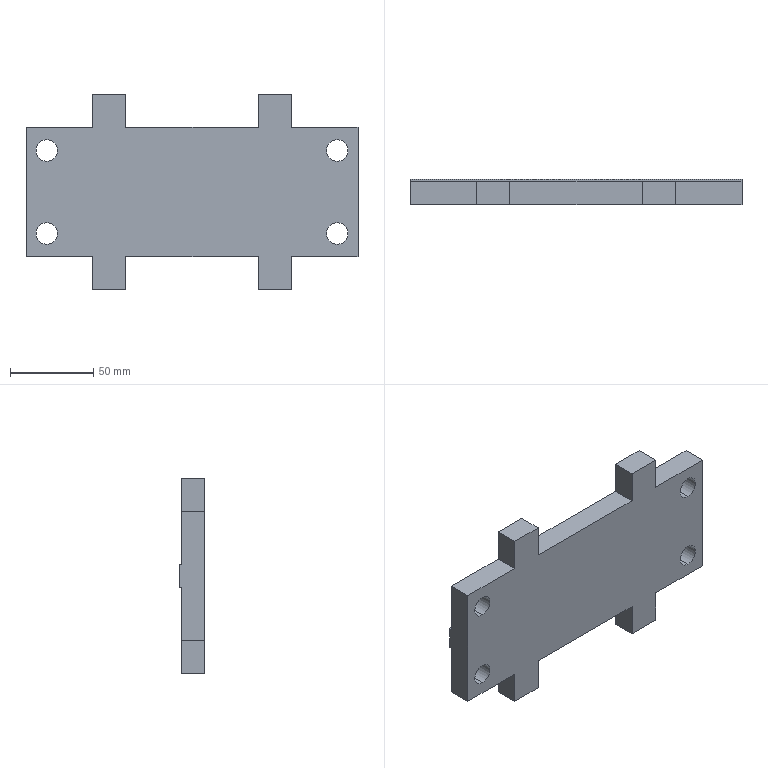Component | SolidWorks | NewTypeCurveBenderReinforcementSeatUpperWheelBox2-DoubleWheel-1 | 1 solid | 34 faces | box 200 x 15.5 x 118 mm | volume 237567 mm3 | plane 26 | cylinder 8 | commonest cylinder face diameters 13 x8
build123d program:
from build123d import *

# Parameters (mm, degrees)
SKETCH1_W           = 200
SKETCH1_H           = 78
BOSS_EXTRUDE1_DEPTH = 14
SKETCH2_W           = 20
SKETCH2_H           = 20
BOSS_EXTRUDE2_DEPTH = 14
SKETCH3_R           = 6.5
CUT_EXTRUDE1_DEPTH  = 30
SKETCH5_W           = 14
SKETCH5_H           = 1.5
BOSS_EXTRUDE3_DEPTH = 200


with BuildPart() as part:
    # Sketch1 → Boss-Extrude1 (new body)
    with BuildSketch(Plane(origin=(0, 0, 0), x_dir=(1, 0, 0), z_dir=(0, 1, 0))):
        Rectangle(SKETCH1_W, SKETCH1_H)
    extrude(amount=BOSS_EXTRUDE1_DEPTH)

    # Sketch2 → Boss-Extrude2 (add)
    with BuildSketch(Plane(origin=(0, 14, 0), x_dir=(1, 0, 0), z_dir=(0, 1, 0))):
        with Locations((-50, -49)):
            Rectangle(SKETCH2_W, SKETCH2_H)
        with Locations((-50, 49)):
            Rectangle(SKETCH2_W, SKETCH2_H)
        with Locations((50, -49)):
            Rectangle(SKETCH2_W, SKETCH2_H)
        with Locations((50, 49)):
            Rectangle(SKETCH2_W, SKETCH2_H)
    extrude(amount=-BOSS_EXTRUDE2_DEPTH)

    # Sketch3 → Cut-Extrude1 (cut)
    with BuildSketch(Plane(origin=(0, 14, 0), x_dir=(1, 0, 0), z_dir=(0, 1, 0))):
        with Locations(Location((-87.5, 25, 0), (0, 0, 270))):
            Circle(SKETCH3_R)
        with Locations(Location((87.5, 25, 0), (0, 0, 270))):
            Circle(SKETCH3_R)
        with Locations(Location((87.5, -25, 0), (0, 0, 270))):
            Circle(SKETCH3_R)
        with Locations(Location((-87.5, -25, 0), (0, 0, 270))):
            Circle(SKETCH3_R)
    extrude(amount=-CUT_EXTRUDE1_DEPTH, mode=Mode.SUBTRACT)

    # Sketch5 → Boss-Extrude3 (add)
    with BuildSketch(Plane(origin=(100, 0, 0), x_dir=(0, 0, -1), z_dir=(1, 0, 0))):
        with Locations((0, -0.75)):
            Rectangle(SKETCH5_W, SKETCH5_H)
    extrude(amount=-BOSS_EXTRUDE3_DEPTH)


solid = part.part

# Placed as in the assembly
solid = solid.moved(Location((0, -133, 0), (180, 0, 0)))
STEP:
#1=COLOUR_RGB('',0.7922,0.8196,0.9333);
#2=FILL_AREA_STYLE_COLOUR('',#1);
#3=FILL_AREA_STYLE('',(#2));
#4=SURFACE_STYLE_FILL_AREA(#3);
#5=SURFACE_SIDE_STYLE('',(#4));
#6=SURFACE_STYLE_USAGE(.BOTH.,#5);
#7=PRESENTATION_STYLE_ASSIGNMENT((#6));
#8=CARTESIAN_POINT('',(3.445,-5.236,0.7283));
#9=VERTEX_POINT('',#8);
#10=CARTESIAN_POINT('',(3.445,-5.236,1.24));
#11=VERTEX_POINT('',#10);
#12=CARTESIAN_POINT('',(3.445,-5.236,0.9843));
#13=DIRECTION('',(0.,-1.,-0.));
#14=DIRECTION('',(0.,0.,1.));
#15=AXIS2_PLACEMENT_3D('',#12,#13,#14);
#16=CIRCLE('',#15,0.2559);
#17=EDGE_CURVE('',#9,#11,#16,.T.);
#18=ORIENTED_EDGE('',*,*,#17,.F.);
#19=CARTESIAN_POINT('',(3.445,-5.787,0.7283));
#20=VERTEX_POINT('',#19);
#21=CARTESIAN_POINT('',(3.445,-4.606,0.7283));
#22=DIRECTION('',(0.,-1.,-0.));
#23=VECTOR('',#22,39.37);
#24=LINE('',#21,#23);
#25=EDGE_CURVE('',#9,#20,#24,.T.);
#26=ORIENTED_EDGE('',*,*,#25,.T.);
#27=CARTESIAN_POINT('',(3.445,-5.787,1.24));
#28=VERTEX_POINT('',#27);
#29=CARTESIAN_POINT('',(3.445,-5.787,0.9843));
#30=DIRECTION('',(0.,-1.,-0.));
#31=DIRECTION('',(0.,0.,-1.));
#32=AXIS2_PLACEMENT_3D('',#29,#30,#31);
#33=CIRCLE('',#32,0.2559);
#34=EDGE_CURVE('',#20,#28,#33,.T.);
#35=ORIENTED_EDGE('',*,*,#34,.T.);
#36=CARTESIAN_POINT('',(3.445,-4.606,1.24));
#37=DIRECTION('',(0.,-1.,-0.));
#38=VECTOR('',#37,39.37);
#39=LINE('',#36,#38);
#40=EDGE_CURVE('',#11,#28,#39,.T.);
#41=ORIENTED_EDGE('',*,*,#40,.F.);
#42=EDGE_LOOP('',(#18,#26,#35,#41));
#43=FACE_OUTER_BOUND('',#42,.T.);
#44=CARTESIAN_POINT('',(3.445,-4.606,0.9843));
#45=DIRECTION('',(0.,-1.,-0.));
#46=DIRECTION('',(0.,0.,1.));
#47=AXIS2_PLACEMENT_3D('',#44,#45,#46);
#48=CYLINDRICAL_SURFACE('',#47,0.2559);
#49=ADVANCED_FACE('',(#43),#48,.F.);
#50=CARTESIAN_POINT('',(-3.445,-5.236,0.7283));
#51=VERTEX_POINT('',#50);
#52=CARTESIAN_POINT('',(-3.445,-5.236,1.24));
#53=VERTEX_POINT('',#52);
#54=CARTESIAN_POINT('',(-3.445,-5.236,0.9843));
#55=DIRECTION('',(0.,-1.,-0.));
#56=DIRECTION('',(0.,0.,1.));
#57=AXIS2_PLACEMENT_3D('',#54,#55,#56);
#58=CIRCLE('',#57,0.2559);
#59=EDGE_CURVE('',#51,#53,#58,.T.);
#60=ORIENTED_EDGE('',*,*,#59,.F.);
#61=CARTESIAN_POINT('',(-3.445,-5.787,0.7283));
#62=VERTEX_POINT('',#61);
#63=CARTESIAN_POINT('',(-3.445,-4.606,0.7283));
#64=DIRECTION('',(0.,-1.,-0.));
#65=VECTOR('',#64,39.37);
#66=LINE('',#63,#65);
#67=EDGE_CURVE('',#51,#62,#66,.T.);
#68=ORIENTED_EDGE('',*,*,#67,.T.);
#69=CARTESIAN_POINT('',(-3.445,-5.787,1.24));
#70=VERTEX_POINT('',#69);
#71=CARTESIAN_POINT('',(-3.445,-5.787,0.9843));
#72=DIRECTION('',(0.,-1.,-0.));
#73=DIRECTION('',(0.,0.,1.));
#74=AXIS2_PLACEMENT_3D('',#71,#72,#73);
#75=CIRCLE('',#74,0.2559);
#76=EDGE_CURVE('',#62,#70,#75,.T.);
#77=ORIENTED_EDGE('',*,*,#76,.T.);
#78=CARTESIAN_POINT('',(-3.445,-4.606,1.24));
#79=DIRECTION('',(0.,-1.,-0.));
#80=VECTOR('',#79,39.37);
#81=LINE('',#78,#80);
#82=EDGE_CURVE('',#53,#70,#81,.T.);
#83=ORIENTED_EDGE('',*,*,#82,.F.);
#84=EDGE_LOOP('',(#60,#68,#77,#83));
#85=FACE_OUTER_BOUND('',#84,.T.);
#86=CARTESIAN_POINT('',(-3.445,-4.606,0.9843));
#87=DIRECTION('',(0.,-1.,-0.));
#88=DIRECTION('',(0.,0.,1.));
#89=AXIS2_PLACEMENT_3D('',#86,#87,#88);
#90=CYLINDRICAL_SURFACE('',#89,0.2559);
#91=ADVANCED_FACE('',(#85),#90,.F.);
#92=CARTESIAN_POINT('',(-3.445,-5.236,-1.24));
#93=VERTEX_POINT('',#92);
#94=CARTESIAN_POINT('',(-3.445,-5.236,-0.7283));
#95=VERTEX_POINT('',#94);
#96=CARTESIAN_POINT('',(-3.445,-5.236,-0.9843));
#97=DIRECTION('',(0.,-1.,-0.));
#98=DIRECTION('',(0.,0.,1.));
#99=AXIS2_PLACEMENT_3D('',#96,#97,#98);
#100=CIRCLE('',#99,0.2559);
#101=EDGE_CURVE('',#93,#95,#100,.T.);
#102=ORIENTED_EDGE('',*,*,#101,.F.);
#103=CARTESIAN_POINT('',(-3.445,-5.787,-1.24));
#104=VERTEX_POINT('',#103);
#105=CARTESIAN_POINT('',(-3.445,-4.606,-1.24));
#106=DIRECTION('',(0.,-1.,-0.));
#107=VECTOR('',#106,39.37);
#108=LINE('',#105,#107);
#109=EDGE_CURVE('',#93,#104,#108,.T.);
#110=ORIENTED_EDGE('',*,*,#109,.T.);
#111=CARTESIAN_POINT('',(-3.445,-5.787,-0.7283));
#112=VERTEX_POINT('',#111);
#113=CARTESIAN_POINT('',(-3.445,-5.787,-0.9843));
#114=DIRECTION('',(0.,-1.,-0.));
#115=DIRECTION('',(0.,0.,-1.));
#116=AXIS2_PLACEMENT_3D('',#113,#114,#115);
#117=CIRCLE('',#116,0.2559);
#118=EDGE_CURVE('',#104,#112,#117,.T.);
#119=ORIENTED_EDGE('',*,*,#118,.T.);
#120=CARTESIAN_POINT('',(-3.445,-4.606,-0.7283));
#121=DIRECTION('',(0.,-1.,-0.));
#122=VECTOR('',#121,39.37);
#123=LINE('',#120,#122);
#124=EDGE_CURVE('',#95,#112,#123,.T.);
#125=ORIENTED_EDGE('',*,*,#124,.F.);
#126=EDGE_LOOP('',(#102,#110,#119,#125));
#127=FACE_OUTER_BOUND('',#126,.T.);
#128=CARTESIAN_POINT('',(-3.445,-4.606,-0.9843));
#129=DIRECTION('',(0.,-1.,-0.));
#130=DIRECTION('',(0.,0.,1.));
#131=AXIS2_PLACEMENT_3D('',#128,#129,#130);
#132=CYLINDRICAL_SURFACE('',#131,0.2559);
#133=ADVANCED_FACE('',(#127),#132,.F.);
#134=CARTESIAN_POINT('',(3.445,-5.236,-1.24));
#135=VERTEX_POINT('',#134);
#136=CARTESIAN_POINT('',(3.445,-5.236,-0.7283));
#137=VERTEX_POINT('',#136);
#138=CARTESIAN_POINT('',(3.445,-5.236,-0.9843));
#139=DIRECTION('',(0.,-1.,-0.));
#140=DIRECTION('',(0.,0.,1.));
#141=AXIS2_PLACEMENT_3D('',#138,#139,#140);
#142=CIRCLE('',#141,0.2559);
#143=EDGE_CURVE('',#135,#137,#142,.T.);
#144=ORIENTED_EDGE('',*,*,#143,.F.);
#145=CARTESIAN_POINT('',(3.445,-5.787,-1.24));
#146=VERTEX_POINT('',#145);
#147=CARTESIAN_POINT('',(3.445,-4.606,-1.24));
#148=DIRECTION('',(0.,-1.,-0.));
#149=VECTOR('',#148,39.37);
#150=LINE('',#147,#149);
#151=EDGE_CURVE('',#135,#146,#150,.T.);
#152=ORIENTED_EDGE('',*,*,#151,.T.);
#153=CARTESIAN_POINT('',(3.445,-5.787,-0.7283));
#154=VERTEX_POINT('',#153);
#155=CARTESIAN_POINT('',(3.445,-5.787,-0.9843));
#156=DIRECTION('',(0.,-1.,-0.));
#157=DIRECTION('',(0.,0.,1.));
#158=AXIS2_PLACEMENT_3D('',#155,#156,#157);
#159=CIRCLE('',#158,0.2559);
#160=EDGE_CURVE('',#146,#154,#159,.T.);
#161=ORIENTED_EDGE('',*,*,#160,.T.);
#162=CARTESIAN_POINT('',(3.445,-4.606,-0.7283));
#163=DIRECTION('',(0.,-1.,-0.));
#164=VECTOR('',#163,39.37);
#165=LINE('',#162,#164);
#166=EDGE_CURVE('',#137,#154,#165,.T.);
#167=ORIENTED_EDGE('',*,*,#166,.F.);
#168=EDGE_LOOP('',(#144,#152,#161,#167));
#169=FACE_OUTER_BOUND('',#168,.T.);
#170=CARTESIAN_POINT('',(3.445,-4.606,-0.9843));
#171=DIRECTION('',(0.,-1.,-0.));
#172=DIRECTION('',(0.,0.,1.));
#173=AXIS2_PLACEMENT_3D('',#170,#171,#172);
#174=CYLINDRICAL_SURFACE('',#173,0.2559);
#175=ADVANCED_FACE('',(#169),#174,.F.);
#176=CARTESIAN_POINT('',(3.445,-5.236,-0.9843));
#177=DIRECTION('',(0.,-1.,-0.));
#178=DIRECTION('',(0.,0.,1.));
#179=AXIS2_PLACEMENT_3D('',#176,#177,#178);
#180=CIRCLE('',#179,0.2559);
#181=EDGE_CURVE('',#137,#135,#180,.T.);
#182=ORIENTED_EDGE('',*,*,#181,.T.);
#183=ORIENTED_EDGE('',*,*,#143,.T.);
#184=EDGE_LOOP('',(#182,#183));
#185=FACE_BOUND('',#184,.T.);
#186=CARTESIAN_POINT('',(-3.445,-5.236,-0.9843));
#187=DIRECTION('',(0.,-1.,-0.));
#188=DIRECTION('',(0.,0.,1.));
#189=AXIS2_PLACEMENT_3D('',#186,#187,#188);
#190=CIRCLE('',#189,0.2559);
#191=EDGE_CURVE('',#95,#93,#190,.T.);
#192=ORIENTED_EDGE('',*,*,#191,.T.);
#193=ORIENTED_EDGE('',*,*,#101,.T.);
#194=EDGE_LOOP('',(#192,#193));
#195=FACE_BOUND('',#194,.T.);
#196=CARTESIAN_POINT('',(3.937,-5.236,-0.2756));
#197=VERTEX_POINT('',#196);
#198=CARTESIAN_POINT('',(-3.937,-5.236,-0.2756));
#199=VERTEX_POINT('',#198);
#200=CARTESIAN_POINT('',(4.491,-5.236,-0.2756));
#201=DIRECTION('',(-1.,-0.,0.));
#202=VECTOR('',#201,39.37);
#203=LINE('',#200,#202);
#204=EDGE_CURVE('',#197,#199,#203,.T.);
#205=ORIENTED_EDGE('',*,*,#204,.F.);
#206=CARTESIAN_POINT('',(3.937,-5.236,-1.535));
#207=VERTEX_POINT('',#206);
#208=CARTESIAN_POINT('',(3.937,-5.236,-1.535));
#209=DIRECTION('',(0.,0.,1.));
#210=VECTOR('',#209,39.37);
#211=LINE('',#208,#210);
#212=EDGE_CURVE('',#207,#197,#211,.T.);
#213=ORIENTED_EDGE('',*,*,#212,.F.);
#214=CARTESIAN_POINT('',(2.362,-5.236,-1.535));
#215=VERTEX_POINT('',#214);
#216=CARTESIAN_POINT('',(3.937,-5.236,-1.535));
#217=DIRECTION('',(1.,0.,0.));
#218=VECTOR('',#217,39.37);
#219=LINE('',#216,#218);
#220=EDGE_CURVE('',#215,#207,#219,.T.);
#221=ORIENTED_EDGE('',*,*,#220,.F.);
#222=CARTESIAN_POINT('',(2.362,-5.236,-2.323));
#223=VERTEX_POINT('',#222);
#224=CARTESIAN_POINT('',(2.362,-5.236,-1.535));
#225=DIRECTION('',(0.,-0.,-1.));
#226=VECTOR('',#225,39.37);
#227=LINE('',#224,#226);
#228=EDGE_CURVE('',#215,#223,#227,.T.);
#229=ORIENTED_EDGE('',*,*,#228,.T.);
#230=CARTESIAN_POINT('',(1.575,-5.236,-2.323));
#231=VERTEX_POINT('',#230);
#232=CARTESIAN_POINT('',(2.362,-5.236,-2.323));
#233=DIRECTION('',(-1.,-0.,0.));
#234=VECTOR('',#233,39.37);
#235=LINE('',#232,#234);
#236=EDGE_CURVE('',#223,#231,#235,.T.);
#237=ORIENTED_EDGE('',*,*,#236,.T.);
#238=CARTESIAN_POINT('',(1.575,-5.236,-1.535));
#239=VERTEX_POINT('',#238);
#240=CARTESIAN_POINT('',(1.575,-5.236,-1.535));
#241=DIRECTION('',(0.,0.,1.));
#242=VECTOR('',#241,39.37);
#243=LINE('',#240,#242);
#244=EDGE_CURVE('',#231,#239,#243,.T.);
#245=ORIENTED_EDGE('',*,*,#244,.T.);
#246=CARTESIAN_POINT('',(-1.575,-5.236,-1.535));
#247=VERTEX_POINT('',#246);
#248=CARTESIAN_POINT('',(3.937,-5.236,-1.535));
#249=DIRECTION('',(1.,0.,0.));
#250=VECTOR('',#249,39.37);
#251=LINE('',#248,#250);
#252=EDGE_CURVE('',#247,#239,#251,.T.);
#253=ORIENTED_EDGE('',*,*,#252,.F.);
#254=CARTESIAN_POINT('',(-1.575,-5.236,-2.323));
#255=VERTEX_POINT('',#254);
#256=CARTESIAN_POINT('',(-1.575,-5.236,-1.535));
#257=DIRECTION('',(-0.,-0.,-1.));
#258=VECTOR('',#257,39.37);
#259=LINE('',#256,#258);
#260=EDGE_CURVE('',#247,#255,#259,.T.);
#261=ORIENTED_EDGE('',*,*,#260,.T.);
#262=CARTESIAN_POINT('',(-2.362,-5.236,-2.323));
#263=VERTEX_POINT('',#262);
#264=CARTESIAN_POINT('',(-2.362,-5.236,-2.323));
#265=DIRECTION('',(-1.,-0.,-0.));
#266=VECTOR('',#265,39.37);
#267=LINE('',#264,#266);
#268=EDGE_CURVE('',#255,#263,#267,.T.);
#269=ORIENTED_EDGE('',*,*,#268,.T.);
#270=CARTESIAN_POINT('',(-2.362,-5.236,-1.535));
#271=VERTEX_POINT('',#270);
#272=CARTESIAN_POINT('',(-2.362,-5.236,-1.535));
#273=DIRECTION('',(0.,0.,1.));
#274=VECTOR('',#273,39.37);
#275=LINE('',#272,#274);
#276=EDGE_CURVE('',#263,#271,#275,.T.);
#277=ORIENTED_EDGE('',*,*,#276,.T.);
#278=CARTESIAN_POINT('',(-3.937,-5.236,-1.535));
#279=VERTEX_POINT('',#278);
#280=CARTESIAN_POINT('',(3.937,-5.236,-1.535));
#281=DIRECTION('',(1.,0.,0.));
#282=VECTOR('',#281,39.37);
#283=LINE('',#280,#282);
#284=EDGE_CURVE('',#279,#271,#283,.T.);
#285=ORIENTED_EDGE('',*,*,#284,.F.);
#286=CARTESIAN_POINT('',(-3.937,-5.236,-1.535));
#287=DIRECTION('',(-0.,-0.,-1.));
#288=VECTOR('',#287,39.37);
#289=LINE('',#286,#288);
#290=EDGE_CURVE('',#199,#279,#289,.T.);
#291=ORIENTED_EDGE('',*,*,#290,.F.);
#292=EDGE_LOOP('',(#205,#213,#221,#229,#237,#245,#253,#261,#269,#277,#285,#291));
#293=FACE_OUTER_BOUND('',#292,.T.);
#294=CARTESIAN_POINT('',(-0.,-5.236,0.));
#295=DIRECTION('',(0.,-1.,0.));
#296=DIRECTION('',(0.,0.,1.));
#297=AXIS2_PLACEMENT_3D('',#294,#295,#296);
#298=PLANE('',#297);
#299=ADVANCED_FACE('',(#185,#195,#293),#298,.F.);
#300=CARTESIAN_POINT('',(-1.575,-5.787,-1.535));
#301=VERTEX_POINT('',#300);
#302=CARTESIAN_POINT('',(1.575,-5.787,-1.535));
#303=VERTEX_POINT('',#302);
#304=CARTESIAN_POINT('',(3.937,-5.787,-1.535));
#305=DIRECTION('',(1.,0.,0.));
#306=VECTOR('',#305,39.37);
#307=LINE('',#304,#306);
#308=EDGE_CURVE('',#301,#303,#307,.T.);
#309=ORIENTED_EDGE('',*,*,#308,.F.);
#310=CARTESIAN_POINT('',(-1.575,-4.123,-1.535));
#311=DIRECTION('',(0.,-1.,-0.));
#312=VECTOR('',#311,39.37);
#313=LINE('',#310,#312);
#314=EDGE_CURVE('',#247,#301,#313,.T.);
#315=ORIENTED_EDGE('',*,*,#314,.F.);
#316=ORIENTED_EDGE('',*,*,#252,.T.);
#317=CARTESIAN_POINT('',(1.575,-4.123,-1.535));
#318=DIRECTION('',(0.,-1.,-0.));
#319=VECTOR('',#318,39.37);
#320=LINE('',#317,#319);
#321=EDGE_CURVE('',#239,#303,#320,.T.);
#322=ORIENTED_EDGE('',*,*,#321,.T.);
#323=EDGE_LOOP('',(#309,#315,#316,#322));
#324=FACE_OUTER_BOUND('',#323,.T.);
#325=CARTESIAN_POINT('',(3.937,-5.787,-1.535));
#326=DIRECTION('',(-0.,0.,1.));
#327=DIRECTION('',(-1.,-0.,0.));
#328=AXIS2_PLACEMENT_3D('',#325,#326,#327);
#329=PLANE('',#328);
#330=ADVANCED_FACE('',(#324),#329,.F.);
#331=CARTESIAN_POINT('',(-2.362,-5.787,1.535));
#332=VERTEX_POINT('',#331);
#333=CARTESIAN_POINT('',(-3.937,-5.787,1.535));
#334=VERTEX_POINT('',#333);
#335=CARTESIAN_POINT('',(3.937,-5.787,1.535));
#336=DIRECTION('',(-1.,-0.,0.));
#337=VECTOR('',#336,39.37);
#338=LINE('',#335,#337);
#339=EDGE_CURVE('',#332,#334,#338,.T.);
#340=ORIENTED_EDGE('',*,*,#339,.F.);
#341=CARTESIAN_POINT('',(-2.362,-5.236,1.535));
#342=VERTEX_POINT('',#341);
#343=CARTESIAN_POINT('',(-2.362,-4.123,1.535));
#344=DIRECTION('',(0.,-1.,-0.));
#345=VECTOR('',#344,39.37);
#346=LINE('',#343,#345);
#347=EDGE_CURVE('',#342,#332,#346,.T.);
#348=ORIENTED_EDGE('',*,*,#347,.F.);
#349=CARTESIAN_POINT('',(-3.937,-5.236,1.535));
#350=VERTEX_POINT('',#349);
#351=CARTESIAN_POINT('',(3.937,-5.236,1.535));
#352=DIRECTION('',(-1.,-0.,0.));
#353=VECTOR('',#352,39.37);
#354=LINE('',#351,#353);
#355=EDGE_CURVE('',#342,#350,#354,.T.);
#356=ORIENTED_EDGE('',*,*,#355,.T.);
#357=CARTESIAN_POINT('',(-3.937,-5.787,1.535));
#358=DIRECTION('',(-0.,1.,0.));
#359=VECTOR('',#358,39.37);
#360=LINE('',#357,#359);
#361=EDGE_CURVE('',#334,#350,#360,.T.);
#362=ORIENTED_EDGE('',*,*,#361,.F.);
#363=EDGE_LOOP('',(#340,#348,#356,#362));
#364=FACE_OUTER_BOUND('',#363,.T.);
#365=CARTESIAN_POINT('',(3.937,-5.787,1.535));
#366=DIRECTION('',(0.,-0.,-1.));
#367=DIRECTION('',(1.,0.,0.));
#368=AXIS2_PLACEMENT_3D('',#365,#366,#367);
#369=PLANE('',#368);
#370=ADVANCED_FACE('',(#364),#369,.F.);
#371=CARTESIAN_POINT('',(1.575,-5.236,1.535));
#372=VERTEX_POINT('',#371);
#373=CARTESIAN_POINT('',(-1.575,-5.236,1.535));
#374=VERTEX_POINT('',#373);
#375=CARTESIAN_POINT('',(3.937,-5.236,1.535));
#376=DIRECTION('',(-1.,-0.,0.));
#377=VECTOR('',#376,39.37);
#378=LINE('',#375,#377);
#379=EDGE_CURVE('',#372,#374,#378,.T.);
#380=ORIENTED_EDGE('',*,*,#379,.T.);
#381=CARTESIAN_POINT('',(-1.575,-5.787,1.535));
#382=VERTEX_POINT('',#381);
#383=CARTESIAN_POINT('',(-1.575,-4.123,1.535));
#384=DIRECTION('',(0.,-1.,-0.));
#385=VECTOR('',#384,39.37);
#386=LINE('',#383,#385);
#387=EDGE_CURVE('',#374,#382,#386,.T.);
#388=ORIENTED_EDGE('',*,*,#387,.T.);
#389=CARTESIAN_POINT('',(1.575,-5.787,1.535));
#390=VERTEX_POINT('',#389);
#391=CARTESIAN_POINT('',(3.937,-5.787,1.535));
#392=DIRECTION('',(-1.,-0.,0.));
#393=VECTOR('',#392,39.37);
#394=LINE('',#391,#393);
#395=EDGE_CURVE('',#390,#382,#394,.T.);
#396=ORIENTED_EDGE('',*,*,#395,.F.);
#397=CARTESIAN_POINT('',(1.575,-4.123,1.535));
#398=DIRECTION('',(0.,-1.,-0.));
#399=VECTOR('',#398,39.37);
#400=LINE('',#397,#399);
#401=EDGE_CURVE('',#372,#390,#400,.T.);
#402=ORIENTED_EDGE('',*,*,#401,.F.);
#403=EDGE_LOOP('',(#380,#388,#396,#402));
#404=FACE_OUTER_BOUND('',#403,.T.);
#405=CARTESIAN_POINT('',(3.937,-5.787,1.535));
#406=DIRECTION('',(0.,-0.,-1.));
#407=DIRECTION('',(1.,0.,0.));
#408=AXIS2_PLACEMENT_3D('',#405,#406,#407);
#409=PLANE('',#408);
#410=ADVANCED_FACE('',(#404),#409,.F.);
#411=CARTESIAN_POINT('',(2.362,-5.787,-1.535));
#412=VERTEX_POINT('',#411);
#413=CARTESIAN_POINT('',(2.362,-4.123,-1.535));
#414=DIRECTION('',(0.,-1.,-0.));
#415=VECTOR('',#414,39.37);
#416=LINE('',#413,#415);
#417=EDGE_CURVE('',#215,#412,#416,.T.);
#418=ORIENTED_EDGE('',*,*,#417,.F.);
#419=ORIENTED_EDGE('',*,*,#220,.T.);
#420=CARTESIAN_POINT('',(3.937,-5.787,-1.535));
#421=VERTEX_POINT('',#420);
#422=CARTESIAN_POINT('',(3.937,-5.787,-1.535));
#423=DIRECTION('',(-0.,1.,0.));
#424=VECTOR('',#423,39.37);
#425=LINE('',#422,#424);
#426=EDGE_CURVE('',#421,#207,#425,.T.);
#427=ORIENTED_EDGE('',*,*,#426,.F.);
#428=CARTESIAN_POINT('',(3.937,-5.787,-1.535));
#429=DIRECTION('',(1.,0.,0.));
#430=VECTOR('',#429,39.37);
#431=LINE('',#428,#430);
#432=EDGE_CURVE('',#412,#421,#431,.T.);
#433=ORIENTED_EDGE('',*,*,#432,.F.);
#434=EDGE_LOOP('',(#418,#419,#427,#433));
#435=FACE_OUTER_BOUND('',#434,.T.);
#436=CARTESIAN_POINT('',(3.937,-5.787,-1.535));
#437=DIRECTION('',(-0.,0.,1.));
#438=DIRECTION('',(-1.,-0.,0.));
#439=AXIS2_PLACEMENT_3D('',#436,#437,#438);
#440=PLANE('',#439);
#441=ADVANCED_FACE('',(#435),#440,.F.);
#442=CARTESIAN_POINT('',(-3.937,-5.236,0.2756));
#443=VERTEX_POINT('',#442);
#444=CARTESIAN_POINT('',(-3.937,-5.236,-1.535));
#445=DIRECTION('',(-0.,-0.,-1.));
#446=VECTOR('',#445,39.37);
#447=LINE('',#444,#446);
#448=EDGE_CURVE('',#350,#443,#447,.T.);
#449=ORIENTED_EDGE('',*,*,#448,.T.);
#450=CARTESIAN_POINT('',(-3.937,-5.177,0.2756));
#451=VERTEX_POINT('',#450);
#452=CARTESIAN_POINT('',(-3.937,-5.236,0.2756));
#453=DIRECTION('',(-0.,1.,-0.));
#454=VECTOR('',#453,39.37);
#455=LINE('',#452,#454);
#456=EDGE_CURVE('',#443,#451,#455,.T.);
#457=ORIENTED_EDGE('',*,*,#456,.T.);
#458=CARTESIAN_POINT('',(-3.937,-5.177,-0.2756));
#459=VERTEX_POINT('',#458);
#460=CARTESIAN_POINT('',(-3.937,-5.177,0.2756));
#461=DIRECTION('',(0.,-0.,-1.));
#462=VECTOR('',#461,39.37);
#463=LINE('',#460,#462);
#464=EDGE_CURVE('',#451,#459,#463,.T.);
#465=ORIENTED_EDGE('',*,*,#464,.T.);
#466=CARTESIAN_POINT('',(-3.937,-5.236,-0.2756));
#467=DIRECTION('',(0.,-1.,-0.));
#468=VECTOR('',#467,39.37);
#469=LINE('',#466,#468);
#470=EDGE_CURVE('',#459,#199,#469,.T.);
#471=ORIENTED_EDGE('',*,*,#470,.T.);
#472=ORIENTED_EDGE('',*,*,#290,.T.);
#473=CARTESIAN_POINT('',(-3.937,-5.787,-1.535));
#474=VERTEX_POINT('',#473);
#475=CARTESIAN_POINT('',(-3.937,-5.787,-1.535));
#476=DIRECTION('',(-0.,1.,0.));
#477=VECTOR('',#476,39.37);
#478=LINE('',#475,#477);
#479=EDGE_CURVE('',#474,#279,#478,.T.);
#480=ORIENTED_EDGE('',*,*,#479,.F.);
#481=CARTESIAN_POINT('',(-3.937,-5.787,-1.535));
#482=DIRECTION('',(-0.,-0.,-1.));
#483=VECTOR('',#482,39.37);
#484=LINE('',#481,#483);
#485=EDGE_CURVE('',#334,#474,#484,.T.);
#486=ORIENTED_EDGE('',*,*,#485,.F.);
#487=ORIENTED_EDGE('',*,*,#361,.T.);
#488=EDGE_LOOP('',(#449,#457,#465,#471,#472,#480,#486,#487));
#489=FACE_OUTER_BOUND('',#488,.T.);
#490=CARTESIAN_POINT('',(-3.937,-5.787,-1.535));
#491=DIRECTION('',(1.,0.,-0.));
#492=DIRECTION('',(0.,0.,1.));
#493=AXIS2_PLACEMENT_3D('',#490,#491,#492);
#494=PLANE('',#493);
#495=ADVANCED_FACE('',(#489),#494,.F.);
#496=ORIENTED_EDGE('',*,*,#284,.T.);
#497=CARTESIAN_POINT('',(-2.362,-5.787,-1.535));
#498=VERTEX_POINT('',#497);
#499=CARTESIAN_POINT('',(-2.362,-4.123,-1.535));
#500=DIRECTION('',(0.,-1.,-0.));
#501=VECTOR('',#500,39.37);
#502=LINE('',#499,#501);
#503=EDGE_CURVE('',#271,#498,#502,.T.);
#504=ORIENTED_EDGE('',*,*,#503,.T.);
#505=CARTESIAN_POINT('',(3.937,-5.787,-1.535));
#506=DIRECTION('',(1.,0.,0.));
#507=VECTOR('',#506,39.37);
#508=LINE('',#505,#507);
#509=EDGE_CURVE('',#474,#498,#508,.T.);
#510=ORIENTED_EDGE('',*,*,#509,.F.);
#511=ORIENTED_EDGE('',*,*,#479,.T.);
#512=EDGE_LOOP('',(#496,#504,#510,#511));
#513=FACE_OUTER_BOUND('',#512,.T.);
#514=CARTESIAN_POINT('',(3.937,-5.787,-1.535));
#515=DIRECTION('',(-0.,0.,1.));
#516=DIRECTION('',(-1.,-0.,0.));
#517=AXIS2_PLACEMENT_3D('',#514,#515,#516);
#518=PLANE('',#517);
#519=ADVANCED_FACE('',(#513),#518,.F.);
#520=ORIENTED_EDGE('',*,*,#212,.T.);
#521=CARTESIAN_POINT('',(3.937,-5.177,-0.2756));
#522=VERTEX_POINT('',#521);
#523=CARTESIAN_POINT('',(3.937,-5.236,-0.2756));
#524=DIRECTION('',(-0.,1.,0.));
#525=VECTOR('',#524,39.37);
#526=LINE('',#523,#525);
#527=EDGE_CURVE('',#197,#522,#526,.T.);
#528=ORIENTED_EDGE('',*,*,#527,.T.);
#529=CARTESIAN_POINT('',(3.937,-5.177,0.2756));
#530=VERTEX_POINT('',#529);
#531=CARTESIAN_POINT('',(3.937,-5.177,0.2756));
#532=DIRECTION('',(0.,0.,1.));
#533=VECTOR('',#532,39.37);
#534=LINE('',#531,#533);
#535=EDGE_CURVE('',#522,#530,#534,.T.);
#536=ORIENTED_EDGE('',*,*,#535,.T.);
#537=CARTESIAN_POINT('',(3.937,-5.236,0.2756));
#538=VERTEX_POINT('',#537);
#539=CARTESIAN_POINT('',(3.937,-5.236,0.2756));
#540=DIRECTION('',(0.,-1.,0.));
#541=VECTOR('',#540,39.37);
#542=LINE('',#539,#541);
#543=EDGE_CURVE('',#530,#538,#542,.T.);
#544=ORIENTED_EDGE('',*,*,#543,.T.);
#545=CARTESIAN_POINT('',(3.937,-5.236,1.535));
#546=VERTEX_POINT('',#545);
#547=CARTESIAN_POINT('',(3.937,-5.236,-1.535));
#548=DIRECTION('',(0.,0.,1.));
#549=VECTOR('',#548,39.37);
#550=LINE('',#547,#549);
#551=EDGE_CURVE('',#538,#546,#550,.T.);
#552=ORIENTED_EDGE('',*,*,#551,.T.);
#553=CARTESIAN_POINT('',(3.937,-5.787,1.535));
#554=VERTEX_POINT('',#553);
#555=CARTESIAN_POINT('',(3.937,-5.787,1.535));
#556=DIRECTION('',(-0.,1.,0.));
#557=VECTOR('',#556,39.37);
#558=LINE('',#555,#557);
#559=EDGE_CURVE('',#554,#546,#558,.T.);
#560=ORIENTED_EDGE('',*,*,#559,.F.);
#561=CARTESIAN_POINT('',(3.937,-5.787,-1.535));
#562=DIRECTION('',(0.,0.,1.));
#563=VECTOR('',#562,39.37);
#564=LINE('',#561,#563);
#565=EDGE_CURVE('',#421,#554,#564,.T.);
#566=ORIENTED_EDGE('',*,*,#565,.F.);
#567=ORIENTED_EDGE('',*,*,#426,.T.);
#568=EDGE_LOOP('',(#520,#528,#536,#544,#552,#560,#566,#567));
#569=FACE_OUTER_BOUND('',#568,.T.);
#570=CARTESIAN_POINT('',(3.937,-5.787,-1.535));
#571=DIRECTION('',(-1.,-0.,0.));
#572=DIRECTION('',(0.,-0.,-1.));
#573=AXIS2_PLACEMENT_3D('',#570,#571,#572);
#574=PLANE('',#573);
#575=ADVANCED_FACE('',(#569),#574,.F.);
#576=CARTESIAN_POINT('',(2.362,-5.236,1.535));
#577=VERTEX_POINT('',#576);
#578=CARTESIAN_POINT('',(3.937,-5.236,1.535));
#579=DIRECTION('',(-1.,-0.,0.));
#580=VECTOR('',#579,39.37);
#581=LINE('',#578,#580);
#582=EDGE_CURVE('',#546,#577,#581,.T.);
#583=ORIENTED_EDGE('',*,*,#582,.T.);
#584=CARTESIAN_POINT('',(2.362,-5.787,1.535));
#585=VERTEX_POINT('',#584);
#586=CARTESIAN_POINT('',(2.362,-4.123,1.535));
#587=DIRECTION('',(0.,-1.,-0.));
#588=VECTOR('',#587,39.37);
#589=LINE('',#586,#588);
#590=EDGE_CURVE('',#577,#585,#589,.T.);
#591=ORIENTED_EDGE('',*,*,#590,.T.);
#592=CARTESIAN_POINT('',(3.937,-5.787,1.535));
#593=DIRECTION('',(-1.,-0.,0.));
#594=VECTOR('',#593,39.37);
#595=LINE('',#592,#594);
#596=EDGE_CURVE('',#554,#585,#595,.T.);
#597=ORIENTED_EDGE('',*,*,#596,.F.);
#598=ORIENTED_EDGE('',*,*,#559,.T.);
#599=EDGE_LOOP('',(#583,#591,#597,#598));
#600=FACE_OUTER_BOUND('',#599,.T.);
#601=CARTESIAN_POINT('',(3.937,-5.787,1.535));
#602=DIRECTION('',(0.,-0.,-1.));
#603=DIRECTION('',(1.,0.,0.));
#604=AXIS2_PLACEMENT_3D('',#601,#602,#603);
#605=PLANE('',#604);
#606=ADVANCED_FACE('',(#600),#605,.F.);
#607=CARTESIAN_POINT('',(3.445,-5.787,0.9843));
#608=DIRECTION('',(0.,-1.,-0.));
#609=DIRECTION('',(0.,0.,-1.));
#610=AXIS2_PLACEMENT_3D('',#607,#608,#609);
#611=CIRCLE('',#610,0.2559);
#612=EDGE_CURVE('',#28,#20,#611,.T.);
#613=ORIENTED_EDGE('',*,*,#612,.F.);
#614=ORIENTED_EDGE('',*,*,#34,.F.);
#615=EDGE_LOOP('',(#613,#614));
#616=FACE_BOUND('',#615,.T.);
#617=CARTESIAN_POINT('',(-3.445,-5.787,0.9843));
#618=DIRECTION('',(0.,-1.,-0.));
#619=DIRECTION('',(0.,0.,1.));
#620=AXIS2_PLACEMENT_3D('',#617,#618,#619);
#621=CIRCLE('',#620,0.2559);
#622=EDGE_CURVE('',#70,#62,#621,.T.);
#623=ORIENTED_EDGE('',*,*,#622,.F.);
#624=ORIENTED_EDGE('',*,*,#76,.F.);
#625=EDGE_LOOP('',(#623,#624));
#626=FACE_BOUND('',#625,.T.);
#627=CARTESIAN_POINT('',(-3.445,-5.787,-0.9843));
#628=DIRECTION('',(0.,-1.,-0.));
#629=DIRECTION('',(0.,0.,-1.));
#630=AXIS2_PLACEMENT_3D('',#627,#628,#629);
#631=CIRCLE('',#630,0.2559);
#632=EDGE_CURVE('',#112,#104,#631,.T.);
#633=ORIENTED_EDGE('',*,*,#632,.F.);
#634=ORIENTED_EDGE('',*,*,#118,.F.);
#635=EDGE_LOOP('',(#633,#634));
#636=FACE_BOUND('',#635,.T.);
#637=CARTESIAN_POINT('',(3.445,-5.787,-0.9843));
#638=DIRECTION('',(0.,-1.,-0.));
#639=DIRECTION('',(0.,0.,1.));
#640=AXIS2_PLACEMENT_3D('',#637,#638,#639);
#641=CIRCLE('',#640,0.2559);
#642=EDGE_CURVE('',#154,#146,#641,.T.);
#643=ORIENTED_EDGE('',*,*,#642,.F.);
#644=ORIENTED_EDGE('',*,*,#160,.F.);
#645=EDGE_LOOP('',(#643,#644));
#646=FACE_BOUND('',#645,.T.);
#647=ORIENTED_EDGE('',*,*,#485,.T.);
#648=ORIENTED_EDGE('',*,*,#509,.T.);
#649=CARTESIAN_POINT('',(-2.362,-5.787,-2.323));
#650=VERTEX_POINT('',#649);
#651=CARTESIAN_POINT('',(-2.362,-5.787,-1.535));
#652=DIRECTION('',(-0.,-0.,-1.));
#653=VECTOR('',#652,39.37);
#654=LINE('',#651,#653);
#655=EDGE_CURVE('',#498,#650,#654,.T.);
#656=ORIENTED_EDGE('',*,*,#655,.T.);
#657=CARTESIAN_POINT('',(-1.575,-5.787,-2.323));
#658=VERTEX_POINT('',#657);
#659=CARTESIAN_POINT('',(-2.362,-5.787,-2.323));
#660=DIRECTION('',(1.,0.,0.));
#661=VECTOR('',#660,39.37);
#662=LINE('',#659,#661);
#663=EDGE_CURVE('',#650,#658,#662,.T.);
#664=ORIENTED_EDGE('',*,*,#663,.T.);
#665=CARTESIAN_POINT('',(-1.575,-5.787,-1.535));
#666=DIRECTION('',(0.,0.,1.));
#667=VECTOR('',#666,39.37);
#668=LINE('',#665,#667);
#669=EDGE_CURVE('',#658,#301,#668,.T.);
#670=ORIENTED_EDGE('',*,*,#669,.T.);
#671=ORIENTED_EDGE('',*,*,#308,.T.);
#672=CARTESIAN_POINT('',(1.575,-5.787,-2.323));
#673=VERTEX_POINT('',#672);
#674=CARTESIAN_POINT('',(1.575,-5.787,-1.535));
#675=DIRECTION('',(0.,-0.,-1.));
#676=VECTOR('',#675,39.37);
#677=LINE('',#674,#676);
#678=EDGE_CURVE('',#303,#673,#677,.T.);
#679=ORIENTED_EDGE('',*,*,#678,.T.);
#680=CARTESIAN_POINT('',(2.362,-5.787,-2.323));
#681=VERTEX_POINT('',#680);
#682=CARTESIAN_POINT('',(2.362,-5.787,-2.323));
#683=DIRECTION('',(1.,0.,-0.));
#684=VECTOR('',#683,39.37);
#685=LINE('',#682,#684);
#686=EDGE_CURVE('',#673,#681,#685,.T.);
#687=ORIENTED_EDGE('',*,*,#686,.T.);
#688=CARTESIAN_POINT('',(2.362,-5.787,-1.535));
#689=DIRECTION('',(-0.,0.,1.));
#690=VECTOR('',#689,39.37);
#691=LINE('',#688,#690);
#692=EDGE_CURVE('',#681,#412,#691,.T.);
#693=ORIENTED_EDGE('',*,*,#692,.T.);
#694=ORIENTED_EDGE('',*,*,#432,.T.);
#695=ORIENTED_EDGE('',*,*,#565,.T.);
#696=ORIENTED_EDGE('',*,*,#596,.T.);
#697=CARTESIAN_POINT('',(2.362,-5.787,2.323));
#698=VERTEX_POINT('',#697);
#699=CARTESIAN_POINT('',(2.362,-5.787,1.535));
#700=DIRECTION('',(0.,0.,1.));
#701=VECTOR('',#700,39.37);
#702=LINE('',#699,#701);
#703=EDGE_CURVE('',#585,#698,#702,.T.);
#704=ORIENTED_EDGE('',*,*,#703,.T.);
#705=CARTESIAN_POINT('',(1.575,-5.787,2.323));
#706=VERTEX_POINT('',#705);
#707=CARTESIAN_POINT('',(2.362,-5.787,2.323));
#708=DIRECTION('',(-1.,-0.,-0.));
#709=VECTOR('',#708,39.37);
#710=LINE('',#707,#709);
#711=EDGE_CURVE('',#698,#706,#710,.T.);
#712=ORIENTED_EDGE('',*,*,#711,.T.);
#713=CARTESIAN_POINT('',(1.575,-5.787,1.535));
#714=DIRECTION('',(0.,-0.,-1.));
#715=VECTOR('',#714,39.37);
#716=LINE('',#713,#715);
#717=EDGE_CURVE('',#706,#390,#716,.T.);
#718=ORIENTED_EDGE('',*,*,#717,.T.);
#719=ORIENTED_EDGE('',*,*,#395,.T.);
#720=CARTESIAN_POINT('',(-1.575,-5.787,2.323));
#721=VERTEX_POINT('',#720);
#722=CARTESIAN_POINT('',(-1.575,-5.787,1.535));
#723=DIRECTION('',(-0.,0.,1.));
#724=VECTOR('',#723,39.37);
#725=LINE('',#722,#724);
#726=EDGE_CURVE('',#382,#721,#725,.T.);
#727=ORIENTED_EDGE('',*,*,#726,.T.);
#728=CARTESIAN_POINT('',(-2.362,-5.787,2.323));
#729=VERTEX_POINT('',#728);
#730=CARTESIAN_POINT('',(-2.362,-5.787,2.323));
#731=DIRECTION('',(-1.,-0.,0.));
#732=VECTOR('',#731,39.37);
#733=LINE('',#730,#732);
#734=EDGE_CURVE('',#721,#729,#733,.T.);
#735=ORIENTED_EDGE('',*,*,#734,.T.);
#736=CARTESIAN_POINT('',(-2.362,-5.787,1.535));
#737=DIRECTION('',(0.,-0.,-1.));
#738=VECTOR('',#737,39.37);
#739=LINE('',#736,#738);
#740=EDGE_CURVE('',#729,#332,#739,.T.);
#741=ORIENTED_EDGE('',*,*,#740,.T.);
#742=ORIENTED_EDGE('',*,*,#339,.T.);
#743=EDGE_LOOP('',(#647,#648,#656,#664,#670,#671,#679,#687,#693,#694,#695,#696,#704,#712,#718,#719,#727,#735,#741,#742));
#744=FACE_OUTER_BOUND('',#743,.T.);
#745=CARTESIAN_POINT('',(-0.,-5.787,0.));
#746=DIRECTION('',(0.,-1.,0.));
#747=DIRECTION('',(0.,0.,1.));
#748=AXIS2_PLACEMENT_3D('',#745,#746,#747);
#749=PLANE('',#748);
#750=ADVANCED_FACE('',(#616,#626,#636,#646,#744),#749,.T.);
#751=CARTESIAN_POINT('',(3.445,-5.236,0.9843));
#752=DIRECTION('',(0.,-1.,-0.));
#753=DIRECTION('',(0.,0.,1.));
#754=AXIS2_PLACEMENT_3D('',#751,#752,#753);
#755=CIRCLE('',#754,0.2559);
#756=EDGE_CURVE('',#11,#9,#755,.T.);
#757=ORIENTED_EDGE('',*,*,#756,.T.);
#758=ORIENTED_EDGE('',*,*,#17,.T.);
#759=EDGE_LOOP('',(#757,#758));
#760=FACE_BOUND('',#759,.T.);
#761=CARTESIAN_POINT('',(-3.445,-5.236,0.9843));
#762=DIRECTION('',(0.,-1.,-0.));
#763=DIRECTION('',(0.,0.,1.));
#764=AXIS2_PLACEMENT_3D('',#761,#762,#763);
#765=CIRCLE('',#764,0.2559);
#766=EDGE_CURVE('',#53,#51,#765,.T.);
#767=ORIENTED_EDGE('',*,*,#766,.T.);
#768=ORIENTED_EDGE('',*,*,#59,.T.);
#769=EDGE_LOOP('',(#767,#768));
#770=FACE_BOUND('',#769,.T.);
#771=ORIENTED_EDGE('',*,*,#551,.F.);
#772=CARTESIAN_POINT('',(4.491,-5.236,0.2756));
#773=DIRECTION('',(-1.,-0.,0.));
#774=VECTOR('',#773,39.37);
#775=LINE('',#772,#774);
#776=EDGE_CURVE('',#538,#443,#775,.T.);
#777=ORIENTED_EDGE('',*,*,#776,.T.);
#778=ORIENTED_EDGE('',*,*,#448,.F.);
#779=ORIENTED_EDGE('',*,*,#355,.F.);
#780=CARTESIAN_POINT('',(-2.362,-5.236,2.323));
#781=VERTEX_POINT('',#780);
#782=CARTESIAN_POINT('',(-2.362,-5.236,1.535));
#783=DIRECTION('',(-0.,0.,1.));
#784=VECTOR('',#783,39.37);
#785=LINE('',#782,#784);
#786=EDGE_CURVE('',#342,#781,#785,.T.);
#787=ORIENTED_EDGE('',*,*,#786,.T.);
#788=CARTESIAN_POINT('',(-1.575,-5.236,2.323));
#789=VERTEX_POINT('',#788);
#790=CARTESIAN_POINT('',(-2.362,-5.236,2.323));
#791=DIRECTION('',(1.,0.,-0.));
#792=VECTOR('',#791,39.37);
#793=LINE('',#790,#792);
#794=EDGE_CURVE('',#781,#789,#793,.T.);
#795=ORIENTED_EDGE('',*,*,#794,.T.);
#796=CARTESIAN_POINT('',(-1.575,-5.236,1.535));
#797=DIRECTION('',(0.,-0.,-1.));
#798=VECTOR('',#797,39.37);
#799=LINE('',#796,#798);
#800=EDGE_CURVE('',#789,#374,#799,.T.);
#801=ORIENTED_EDGE('',*,*,#800,.T.);
#802=ORIENTED_EDGE('',*,*,#379,.F.);
#803=CARTESIAN_POINT('',(1.575,-5.236,2.323));
#804=VERTEX_POINT('',#803);
#805=CARTESIAN_POINT('',(1.575,-5.236,1.535));
#806=DIRECTION('',(0.,0.,1.));
#807=VECTOR('',#806,39.37);
#808=LINE('',#805,#807);
#809=EDGE_CURVE('',#372,#804,#808,.T.);
#810=ORIENTED_EDGE('',*,*,#809,.T.);
#811=CARTESIAN_POINT('',(2.362,-5.236,2.323));
#812=VERTEX_POINT('',#811);
#813=CARTESIAN_POINT('',(2.362,-5.236,2.323));
#814=DIRECTION('',(1.,0.,0.));
#815=VECTOR('',#814,39.37);
#816=LINE('',#813,#815);
#817=EDGE_CURVE('',#804,#812,#816,.T.);
#818=ORIENTED_EDGE('',*,*,#817,.T.);
#819=CARTESIAN_POINT('',(2.362,-5.236,1.535));
#820=DIRECTION('',(-0.,-0.,-1.));
#821=VECTOR('',#820,39.37);
#822=LINE('',#819,#821);
#823=EDGE_CURVE('',#812,#577,#822,.T.);
#824=ORIENTED_EDGE('',*,*,#823,.T.);
#825=ORIENTED_EDGE('',*,*,#582,.F.);
#826=EDGE_LOOP('',(#771,#777,#778,#779,#787,#795,#801,#802,#810,#818,#824,#825));
#827=FACE_OUTER_BOUND('',#826,.T.);
#828=CARTESIAN_POINT('',(-0.,-5.236,0.));
#829=DIRECTION('',(0.,-1.,0.));
#830=DIRECTION('',(0.,0.,1.));
#831=AXIS2_PLACEMENT_3D('',#828,#829,#830);
#832=PLANE('',#831);
#833=ADVANCED_FACE('',(#760,#770,#827),#832,.F.);
#834=ORIENTED_EDGE('',*,*,#228,.F.);
#835=ORIENTED_EDGE('',*,*,#417,.T.);
#836=ORIENTED_EDGE('',*,*,#692,.F.);
#837=CARTESIAN_POINT('',(2.362,-4.123,-2.323));
#838=DIRECTION('',(0.,-1.,-0.));
#839=VECTOR('',#838,39.37);
#840=LINE('',#837,#839);
#841=EDGE_CURVE('',#223,#681,#840,.T.);
#842=ORIENTED_EDGE('',*,*,#841,.F.);
#843=EDGE_LOOP('',(#834,#835,#836,#842));
#844=FACE_OUTER_BOUND('',#843,.T.);
#845=CARTESIAN_POINT('',(2.362,-4.123,-1.535));
#846=DIRECTION('',(1.,0.,0.));
#847=DIRECTION('',(-0.,0.,1.));
#848=AXIS2_PLACEMENT_3D('',#845,#846,#847);
#849=PLANE('',#848);
#850=ADVANCED_FACE('',(#844),#849,.T.);
#851=ORIENTED_EDGE('',*,*,#236,.F.);
#852=ORIENTED_EDGE('',*,*,#841,.T.);
#853=ORIENTED_EDGE('',*,*,#686,.F.);
#854=CARTESIAN_POINT('',(1.575,-4.123,-2.323));
#855=DIRECTION('',(0.,-1.,-0.));
#856=VECTOR('',#855,39.37);
#857=LINE('',#854,#856);
#858=EDGE_CURVE('',#231,#673,#857,.T.);
#859=ORIENTED_EDGE('',*,*,#858,.F.);
#860=EDGE_LOOP('',(#851,#852,#853,#859));
#861=FACE_OUTER_BOUND('',#860,.T.);
#862=CARTESIAN_POINT('',(2.362,-4.123,-2.323));
#863=DIRECTION('',(-0.,-0.,-1.));
#864=DIRECTION('',(1.,0.,-0.));
#865=AXIS2_PLACEMENT_3D('',#862,#863,#864);
#866=PLANE('',#865);
#867=ADVANCED_FACE('',(#861),#866,.T.);
#868=ORIENTED_EDGE('',*,*,#244,.F.);
#869=ORIENTED_EDGE('',*,*,#858,.T.);
#870=ORIENTED_EDGE('',*,*,#678,.F.);
#871=ORIENTED_EDGE('',*,*,#321,.F.);
#872=EDGE_LOOP('',(#868,#869,#870,#871));
#873=FACE_OUTER_BOUND('',#872,.T.);
#874=CARTESIAN_POINT('',(1.575,-4.123,-1.535));
#875=DIRECTION('',(-1.,-0.,0.));
#876=DIRECTION('',(0.,-0.,-1.));
#877=AXIS2_PLACEMENT_3D('',#874,#875,#876);
#878=PLANE('',#877);
#879=ADVANCED_FACE('',(#873),#878,.T.);
#880=ORIENTED_EDGE('',*,*,#823,.F.);
#881=CARTESIAN_POINT('',(2.362,-4.123,2.323));
#882=DIRECTION('',(0.,-1.,-0.));
#883=VECTOR('',#882,39.37);
#884=LINE('',#881,#883);
#885=EDGE_CURVE('',#812,#698,#884,.T.);
#886=ORIENTED_EDGE('',*,*,#885,.T.);
#887=ORIENTED_EDGE('',*,*,#703,.F.);
#888=ORIENTED_EDGE('',*,*,#590,.F.);
#889=EDGE_LOOP('',(#880,#886,#887,#888));
#890=FACE_OUTER_BOUND('',#889,.T.);
#891=CARTESIAN_POINT('',(2.362,-4.123,1.535));
#892=DIRECTION('',(1.,0.,-0.));
#893=DIRECTION('',(0.,0.,1.));
#894=AXIS2_PLACEMENT_3D('',#891,#892,#893);
#895=PLANE('',#894);
#896=ADVANCED_FACE('',(#890),#895,.T.);
#897=ORIENTED_EDGE('',*,*,#809,.F.);
#898=ORIENTED_EDGE('',*,*,#401,.T.);
#899=ORIENTED_EDGE('',*,*,#717,.F.);
#900=CARTESIAN_POINT('',(1.575,-4.123,2.323));
#901=DIRECTION('',(0.,-1.,-0.));
#902=VECTOR('',#901,39.37);
#903=LINE('',#900,#902);
#904=EDGE_CURVE('',#804,#706,#903,.T.);
#905=ORIENTED_EDGE('',*,*,#904,.F.);
#906=EDGE_LOOP('',(#897,#898,#899,#905));
#907=FACE_OUTER_BOUND('',#906,.T.);
#908=CARTESIAN_POINT('',(1.575,-4.123,1.535));
#909=DIRECTION('',(-1.,-0.,0.));
#910=DIRECTION('',(0.,-0.,-1.));
#911=AXIS2_PLACEMENT_3D('',#908,#909,#910);
#912=PLANE('',#911);
#913=ADVANCED_FACE('',(#907),#912,.T.);
#914=ORIENTED_EDGE('',*,*,#817,.F.);
#915=ORIENTED_EDGE('',*,*,#904,.T.);
#916=ORIENTED_EDGE('',*,*,#711,.F.);
#917=ORIENTED_EDGE('',*,*,#885,.F.);
#918=EDGE_LOOP('',(#914,#915,#916,#917));
#919=FACE_OUTER_BOUND('',#918,.T.);
#920=CARTESIAN_POINT('',(2.362,-4.123,2.323));
#921=DIRECTION('',(-0.,0.,1.));
#922=DIRECTION('',(-1.,-0.,-0.));
#923=AXIS2_PLACEMENT_3D('',#920,#921,#922);
#924=PLANE('',#923);
#925=ADVANCED_FACE('',(#919),#924,.T.);
#926=ORIENTED_EDGE('',*,*,#786,.F.);
#927=ORIENTED_EDGE('',*,*,#347,.T.);
#928=ORIENTED_EDGE('',*,*,#740,.F.);
#929=CARTESIAN_POINT('',(-2.362,-4.123,2.323));
#930=DIRECTION('',(0.,-1.,-0.));
#931=VECTOR('',#930,39.37);
#932=LINE('',#929,#931);
#933=EDGE_CURVE('',#781,#729,#932,.T.);
#934=ORIENTED_EDGE('',*,*,#933,.F.);
#935=EDGE_LOOP('',(#926,#927,#928,#934));
#936=FACE_OUTER_BOUND('',#935,.T.);
#937=CARTESIAN_POINT('',(-2.362,-4.123,1.535));
#938=DIRECTION('',(-1.,-0.,-0.));
#939=DIRECTION('',(0.,-0.,-1.));
#940=AXIS2_PLACEMENT_3D('',#937,#938,#939);
#941=PLANE('',#940);
#942=ADVANCED_FACE('',(#936),#941,.T.);
#943=ORIENTED_EDGE('',*,*,#794,.F.);
#944=ORIENTED_EDGE('',*,*,#933,.T.);
#945=ORIENTED_EDGE('',*,*,#734,.F.);
#946=CARTESIAN_POINT('',(-1.575,-4.123,2.323));
#947=DIRECTION('',(0.,-1.,-0.));
#948=VECTOR('',#947,39.37);
#949=LINE('',#946,#948);
#950=EDGE_CURVE('',#789,#721,#949,.T.);
#951=ORIENTED_EDGE('',*,*,#950,.F.);
#952=EDGE_LOOP('',(#943,#944,#945,#951));
#953=FACE_OUTER_BOUND('',#952,.T.);
#954=CARTESIAN_POINT('',(-2.362,-4.123,2.323));
#955=DIRECTION('',(0.,0.,1.));
#956=DIRECTION('',(-1.,-0.,0.));
#957=AXIS2_PLACEMENT_3D('',#954,#955,#956);
#958=PLANE('',#957);
#959=ADVANCED_FACE('',(#953),#958,.T.);
#960=ORIENTED_EDGE('',*,*,#800,.F.);
#961=ORIENTED_EDGE('',*,*,#950,.T.);
#962=ORIENTED_EDGE('',*,*,#726,.F.);
#963=ORIENTED_EDGE('',*,*,#387,.F.);
#964=EDGE_LOOP('',(#960,#961,#962,#963));
#965=FACE_OUTER_BOUND('',#964,.T.);
#966=CARTESIAN_POINT('',(-1.575,-4.123,1.535));
#967=DIRECTION('',(1.,0.,0.));
#968=DIRECTION('',(-0.,0.,1.));
#969=AXIS2_PLACEMENT_3D('',#966,#967,#968);
#970=PLANE('',#969);
#971=ADVANCED_FACE('',(#965),#970,.T.);
#972=ORIENTED_EDGE('',*,*,#260,.F.);
#973=ORIENTED_EDGE('',*,*,#314,.T.);
#974=ORIENTED_EDGE('',*,*,#669,.F.);
#975=CARTESIAN_POINT('',(-1.575,-4.123,-2.323));
#976=DIRECTION('',(0.,-1.,-0.));
#977=VECTOR('',#976,39.37);
#978=LINE('',#975,#977);
#979=EDGE_CURVE('',#255,#658,#978,.T.);
#980=ORIENTED_EDGE('',*,*,#979,.F.);
#981=EDGE_LOOP('',(#972,#973,#974,#980));
#982=FACE_OUTER_BOUND('',#981,.T.);
#983=CARTESIAN_POINT('',(-1.575,-4.123,-1.535));
#984=DIRECTION('',(1.,0.,-0.));
#985=DIRECTION('',(0.,0.,1.));
#986=AXIS2_PLACEMENT_3D('',#983,#984,#985);
#987=PLANE('',#986);
#988=ADVANCED_FACE('',(#982),#987,.T.);
#989=ORIENTED_EDGE('',*,*,#268,.F.);
#990=ORIENTED_EDGE('',*,*,#979,.T.);
#991=ORIENTED_EDGE('',*,*,#663,.F.);
#992=CARTESIAN_POINT('',(-2.362,-4.123,-2.323));
#993=DIRECTION('',(0.,-1.,-0.));
#994=VECTOR('',#993,39.37);
#995=LINE('',#992,#994);
#996=EDGE_CURVE('',#263,#650,#995,.T.);
#997=ORIENTED_EDGE('',*,*,#996,.F.);
#998=EDGE_LOOP('',(#989,#990,#991,#997));
#999=FACE_OUTER_BOUND('',#998,.T.);
#1000=CARTESIAN_POINT('',(-2.362,-4.123,-2.323));
#1001=DIRECTION('',(0.,-0.,-1.));
#1002=DIRECTION('',(1.,0.,0.));
#1003=AXIS2_PLACEMENT_3D('',#1000,#1001,#1002);
#1004=PLANE('',#1003);
#1005=ADVANCED_FACE('',(#999),#1004,.T.);
#1006=ORIENTED_EDGE('',*,*,#276,.F.);
#1007=ORIENTED_EDGE('',*,*,#996,.T.);
#1008=ORIENTED_EDGE('',*,*,#655,.F.);
#1009=ORIENTED_EDGE('',*,*,#503,.F.);
#1010=EDGE_LOOP('',(#1006,#1007,#1008,#1009));
#1011=FACE_OUTER_BOUND('',#1010,.T.);
#1012=CARTESIAN_POINT('',(-2.362,-4.123,-1.535));
#1013=DIRECTION('',(-1.,-0.,0.));
#1014=DIRECTION('',(-0.,-0.,-1.));
#1015=AXIS2_PLACEMENT_3D('',#1012,#1013,#1014);
#1016=PLANE('',#1015);
#1017=ADVANCED_FACE('',(#1011),#1016,.T.);
#1018=ORIENTED_EDGE('',*,*,#151,.F.);
#1019=ORIENTED_EDGE('',*,*,#181,.F.);
#1020=ORIENTED_EDGE('',*,*,#166,.T.);
#1021=ORIENTED_EDGE('',*,*,#642,.T.);
#1022=EDGE_LOOP('',(#1018,#1019,#1020,#1021));
#1023=FACE_OUTER_BOUND('',#1022,.T.);
#1024=CARTESIAN_POINT('',(3.445,-4.606,-0.9843));
#1025=DIRECTION('',(0.,-1.,-0.));
#1026=DIRECTION('',(0.,0.,1.));
#1027=AXIS2_PLACEMENT_3D('',#1024,#1025,#1026);
#1028=CYLINDRICAL_SURFACE('',#1027,0.2559);
#1029=ADVANCED_FACE('',(#1023),#1028,.F.);
#1030=ORIENTED_EDGE('',*,*,#109,.F.);
#1031=ORIENTED_EDGE('',*,*,#191,.F.);
#1032=ORIENTED_EDGE('',*,*,#124,.T.);
#1033=ORIENTED_EDGE('',*,*,#632,.T.);
#1034=EDGE_LOOP('',(#1030,#1031,#1032,#1033));
#1035=FACE_OUTER_BOUND('',#1034,.T.);
#1036=CARTESIAN_POINT('',(-3.445,-4.606,-0.9843));
#1037=DIRECTION('',(0.,-1.,-0.));
#1038=DIRECTION('',(0.,0.,1.));
#1039=AXIS2_PLACEMENT_3D('',#1036,#1037,#1038);
#1040=CYLINDRICAL_SURFACE('',#1039,0.2559);
#1041=ADVANCED_FACE('',(#1035),#1040,.F.);
#1042=ORIENTED_EDGE('',*,*,#67,.F.);
#1043=ORIENTED_EDGE('',*,*,#766,.F.);
#1044=ORIENTED_EDGE('',*,*,#82,.T.);
#1045=ORIENTED_EDGE('',*,*,#622,.T.);
#1046=EDGE_LOOP('',(#1042,#1043,#1044,#1045));
#1047=FACE_OUTER_BOUND('',#1046,.T.);
#1048=CARTESIAN_POINT('',(-3.445,-4.606,0.9843));
#1049=DIRECTION('',(0.,-1.,-0.));
#1050=DIRECTION('',(0.,0.,1.));
#1051=AXIS2_PLACEMENT_3D('',#1048,#1049,#1050);
#1052=CYLINDRICAL_SURFACE('',#1051,0.2559);
#1053=ADVANCED_FACE('',(#1047),#1052,.F.);
#1054=ORIENTED_EDGE('',*,*,#25,.F.);
#1055=ORIENTED_EDGE('',*,*,#756,.F.);
#1056=ORIENTED_EDGE('',*,*,#40,.T.);
#1057=ORIENTED_EDGE('',*,*,#612,.T.);
#1058=EDGE_LOOP('',(#1054,#1055,#1056,#1057));
#1059=FACE_OUTER_BOUND('',#1058,.T.);
#1060=CARTESIAN_POINT('',(3.445,-4.606,0.9843));
#1061=DIRECTION('',(0.,-1.,-0.));
#1062=DIRECTION('',(0.,0.,1.));
#1063=AXIS2_PLACEMENT_3D('',#1060,#1061,#1062);
#1064=CYLINDRICAL_SURFACE('',#1063,0.2559);
#1065=ADVANCED_FACE('',(#1059),#1064,.F.);
#1066=ORIENTED_EDGE('',*,*,#527,.F.);
#1067=ORIENTED_EDGE('',*,*,#204,.T.);
#1068=ORIENTED_EDGE('',*,*,#470,.F.);
#1069=CARTESIAN_POINT('',(4.491,-5.177,-0.2756));
#1070=DIRECTION('',(-1.,-0.,0.));
#1071=VECTOR('',#1070,39.37);
#1072=LINE('',#1069,#1071);
#1073=EDGE_CURVE('',#522,#459,#1072,.T.);
#1074=ORIENTED_EDGE('',*,*,#1073,.F.);
#1075=EDGE_LOOP('',(#1066,#1067,#1068,#1074));
#1076=FACE_OUTER_BOUND('',#1075,.T.);
#1077=CARTESIAN_POINT('',(4.491,-5.236,-0.2756));
#1078=DIRECTION('',(-0.,-0.,-1.));
#1079=DIRECTION('',(1.,0.,-0.));
#1080=AXIS2_PLACEMENT_3D('',#1077,#1078,#1079);
#1081=PLANE('',#1080);
#1082=ADVANCED_FACE('',(#1076),#1081,.T.);
#1083=ORIENTED_EDGE('',*,*,#535,.F.);
#1084=ORIENTED_EDGE('',*,*,#1073,.T.);
#1085=ORIENTED_EDGE('',*,*,#464,.F.);
#1086=CARTESIAN_POINT('',(4.491,-5.177,0.2756));
#1087=DIRECTION('',(-1.,-0.,0.));
#1088=VECTOR('',#1087,39.37);
#1089=LINE('',#1086,#1088);
#1090=EDGE_CURVE('',#530,#451,#1089,.T.);
#1091=ORIENTED_EDGE('',*,*,#1090,.F.);
#1092=EDGE_LOOP('',(#1083,#1084,#1085,#1091));
#1093=FACE_OUTER_BOUND('',#1092,.T.);
#1094=CARTESIAN_POINT('',(4.491,-5.177,0.2756));
#1095=DIRECTION('',(-0.,1.,-0.));
#1096=DIRECTION('',(0.,-0.,-1.));
#1097=AXIS2_PLACEMENT_3D('',#1094,#1095,#1096);
#1098=PLANE('',#1097);
#1099=ADVANCED_FACE('',(#1093),#1098,.T.);
#1100=ORIENTED_EDGE('',*,*,#543,.F.);
#1101=ORIENTED_EDGE('',*,*,#1090,.T.);
#1102=ORIENTED_EDGE('',*,*,#456,.F.);
#1103=ORIENTED_EDGE('',*,*,#776,.F.);
#1104=EDGE_LOOP('',(#1100,#1101,#1102,#1103));
#1105=FACE_OUTER_BOUND('',#1104,.T.);
#1106=CARTESIAN_POINT('',(4.491,-5.236,0.2756));
#1107=DIRECTION('',(0.,0.,1.));
#1108=DIRECTION('',(-0.,1.,-0.));
#1109=AXIS2_PLACEMENT_3D('',#1106,#1107,#1108);
#1110=PLANE('',#1109);
#1111=ADVANCED_FACE('',(#1105),#1110,.T.);
#1112=CLOSED_SHELL('',(#49,#91,#133,#175,#299,#330,#370,#410,#441,#495,#519,#575,#606,#750,#833,#850,#867,#879,#896,#913,#925,#942,#959,#971,#988,#1005,#1017,#1029,#1041,#1053,#1065,#1082,#1099,#1111));
#1113=MANIFOLD_SOLID_BREP('',#1112);
#1114=STYLED_ITEM('',(#7),#1113);
#1115=PRESENTATION_LAYER_ASSIGNMENT('','',(#1114));
#1116=(LENGTH_UNIT()NAMED_UNIT(*)SI_UNIT($,.METRE.));
#1117=LENGTH_MEASURE_WITH_UNIT(LENGTH_MEASURE(0.0254),#1116);
#1118=DIMENSIONAL_EXPONENTS(1.,0.,0.,0.,0.,0.,0.);
#1119=(CONVERSION_BASED_UNIT('',#1117)LENGTH_UNIT()NAMED_UNIT(#1118));
#1120=UNCERTAINTY_MEASURE_WITH_UNIT(LENGTH_MEASURE(0.00001),#1119,'','');
#1121=(NAMED_UNIT(*)PLANE_ANGLE_UNIT()SI_UNIT($,.RADIAN.));
#1122=(NAMED_UNIT(*)SI_UNIT($,.STERADIAN.)SOLID_ANGLE_UNIT());
#1123=(GEOMETRIC_REPRESENTATION_CONTEXT(3)GLOBAL_UNCERTAINTY_ASSIGNED_CONTEXT((#1120))GLOBAL_UNIT_ASSIGNED_CONTEXT((#1119,#1121,#1122))REPRESENTATION_CONTEXT('',''));
#1124=MECHANICAL_DESIGN_GEOMETRIC_PRESENTATION_REPRESENTATION('',(#1114),#1123);
#1125=CARTESIAN_POINT('',(0.,0.,0.));
#1126=DIRECTION('',(0.,0.,1.));
#1127=DIRECTION('',(1.,0.,0.));
#1128=AXIS2_PLACEMENT_3D('',#1125,#1126,#1127);
#1129=(LENGTH_UNIT()NAMED_UNIT(*)SI_UNIT($,.METRE.));
#1130=LENGTH_MEASURE_WITH_UNIT(LENGTH_MEASURE(0.0254),#1129);
#1131=DIMENSIONAL_EXPONENTS(1.,0.,0.,0.,0.,0.,0.);
#1132=(CONVERSION_BASED_UNIT('',#1130)LENGTH_UNIT()NAMED_UNIT(#1131));
#1133=UNCERTAINTY_MEASURE_WITH_UNIT(LENGTH_MEASURE(0.00001),#1132,'','');
#1134=(NAMED_UNIT(*)PLANE_ANGLE_UNIT()SI_UNIT($,.RADIAN.));
#1135=(NAMED_UNIT(*)SI_UNIT($,.STERADIAN.)SOLID_ANGLE_UNIT());
#1136=(GEOMETRIC_REPRESENTATION_CONTEXT(3)GLOBAL_UNCERTAINTY_ASSIGNED_CONTEXT((#1133))GLOBAL_UNIT_ASSIGNED_CONTEXT((#1132,#1134,#1135))REPRESENTATION_CONTEXT('',''));
#1137=ADVANCED_BREP_SHAPE_REPRESENTATION('',(#1113,#1128),#1136);